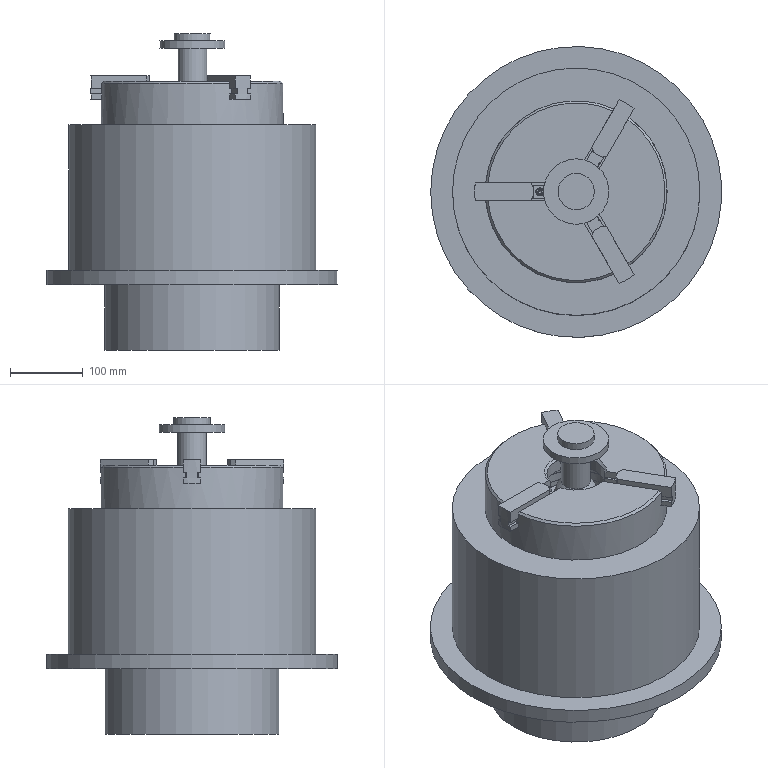Assembly | NX | mm | 45 component files | 45 solids | 1209 faces | box 400 x 400 x 435.36 mm | volume 17965879 mm3 | plane 635 | cone 295 | cylinder 211 | torus 64 | sphere 2 | spline 1 | other 1 | commonest cylinder face diameters 5 x24 6.619 x16 13 x16 6.8 x16 9 x16 15 x16 4.891 x16 10 x16
Bill of materials:
unnamed part 1 | 1 |  | Hollow cylindrical tube with a single wide, thin circular flange around it, set toward one end; the flange has a ring of evenly spaced holes.
GB-T70.1-2000,M8x20 | 8 |  | Hexagon Socket Head Cap Screw, GB-T 70.1-2000,M8x20
unnamed part 2 | 1 |  | Solid stepped round pin: a small boss on top, a thin wide flange, a short neck, a larger cylindrical body, and a smaller end step at the bottom.
unnamed part 3 | 1 |  | Flat circular plate with a large central through hole, an outer ring of 8 holes, an inner ring of 8 smaller holes, and a shallow narrower step (spigot) on one face.
unnamed part 4 | 1 |  | Flanged cup-shaped housing: a wide circular flange, a raised ring on its top face, a cylindrical body below, and a recessed pocket whose floor has a smaller central through hole and several small holes.
unnamed part 5 | 1 |  | Stepped cylinder: a large cylindrical base and a smaller top boss. The boss has a central bore and three radial slots spaced about 120 degrees apart that run from the bore out to the boss edge.
unnamed part 6 | 1 |  | Plain flat ring with a rectangular cross-section, shaped like a washer.
GB-T70.1-2000,M6x25 | 8 |  | Hexagon Socket Head Cap Screw, GB-T 70.1-2000,M6x25
GB-T70.1-2000,M6x20 | 8 |  | Hexagon Socket Head Cap Screw, GB-T 70.1-2000,M6x20
unnamed part 7 | 1 |  | Thick circular disc with a central through bore, a ring of 8 through holes, and a low raised ring around the bore on one face.
unnamed part 8 | 1 |  | Ring with a slightly stepped outer surface; its top face has narrow arc-shaped grooves that look concentric or spiral and end openly.
unnamed part 9 | 1 |  | Round part with a sphere at one end, a cylindrical shank, a thin wide flange, and a short cylindrical boss at the other end.
unnamed part 10 | 1 |  | Headed round part: a larger cylindrical head with a recess that tapers or curves down to a small central hole, on top of a narrower smooth cylindrical shank.
GB-T70.1-2000,M8x60 | 8 |  | Hexagon Socket Head Cap Screw, GB-T 70.1-2000,M8x60
unnamed part 11 | 3 |  | Long prismatic block with a grooved (I- or H-like) cross-section. One end is curved as an arc; the other end has chamfered corners.
Mates:
1. concentric | drag_plate 1 edge | chuck 1 edge
2. concentric | ball_base 1 edge | chuck 1 edge
3. concentric | force_sensor 1 edge | ball_base 1 edge
4. concentric | support_base 1 edge | force_sensor 1 edge
5. concentric | sensor_plate 1 edge | ball_base 1 edge
6. concentric | linear_bearing 1 edge | sensor_plate 1 edge
7. concentric | ball_socket 1 edge | support_base 1 edge
8. touch align | jaw 3 face | chuck 1 face
9. center | jaw 3 face | jaw 3 face | chuck 1 face | chuck 1 face
10. bond | chuck 1 component | assembly component
11. bond | jaw 3 component | assembly component
12. bond | jaw 2 component | assembly component
13. bond | jaw 1 component | assembly component
14. circular | assembly datumaxis | assembly cartesiancoordinatesystem | assembly cartesiancoordinatesystem | assembly cartesiancoordinatesystem
15. concentric | screw_plate 1 edge | chuck 1 edge
16. touch align | ball_mount 1 face | ball_socket 1 face
17. bond | ball_base 1 component | assembly component
18. bond | screw_m8x20 8 component | assembly component
19. bond | screw_m8x20 7 component | assembly component
20. bond | screw_m8x20 6 component | assembly component
21. circular | assembly datumaxis | assembly cartesiancoordinatesystem | assembly cartesiancoordinatesystem | assembly cartesiancoordinatesystem | assembly cartesiancoordinatesystem | assembly cartesiancoordinatesystem | assembly cartesiancoordinatesystem | assembly cartesiancoordinatesystem | assembly cartesiancoordinatesystem
22. bond | screw_m8x20 5 component | assembly component
23. bond | screw_m8x20 4 component | assembly component
24. bond | screw_m8x20 3 component | assembly component
25. bond | screw_m8x20 2 component | assembly component
26. bond | screw_m8x20 1 component | assembly component
27. bond | sensor_plate 1 component | assembly component
28. bond | screw_m6x20 8 component | assembly component
29. bond | screw_m6x20 7 component | assembly component
30. bond | screw_m6x20 6 component | assembly component
31. bond | screw_m6x20 5 component | assembly component
32. bond | screw_m6x20 4 component | assembly component
33. bond | screw_m6x20 3 component | assembly component
34. bond | screw_m6x20 2 component | assembly component
35. bond | screw_m6x20 1 component | assembly component
36. circular | assembly datumaxis | assembly cartesiancoordinatesystem | assembly cartesiancoordinatesystem | assembly cartesiancoordinatesystem | assembly cartesiancoordinatesystem | assembly cartesiancoordinatesystem | assembly cartesiancoordinatesystem | assembly cartesiancoordinatesystem | assembly cartesiancoordinatesystem
37. bond | linear_bearing 1 component | assembly component
38. bond | screw_m6x25 8 component | assembly component
39. bond | screw_m6x25 7 component | assembly component
40. bond | screw_m6x25 6 component | assembly component
41. bond | screw_m6x25 5 component | assembly component
42. bond | screw_m6x25 4 component | assembly component
43. bond | screw_m6x25 3 component | assembly component
44. bond | screw_m6x25 2 component | assembly component
45. bond | screw_m6x25 1 component | assembly component
46. circular | assembly datumaxis | assembly cartesiancoordinatesystem | assembly cartesiancoordinatesystem | assembly cartesiancoordinatesystem | assembly cartesiancoordinatesystem | assembly cartesiancoordinatesystem | assembly cartesiancoordinatesystem | assembly cartesiancoordinatesystem | assembly cartesiancoordinatesystem
47. bond | support_base 1 component | assembly component
48. bond | screw_m8x60 8 component | assembly component
49. bond | screw_m8x60 7 component | assembly component
50. bond | screw_m8x60 6 component | assembly component
51. bond | screw_m8x60 5 component | assembly component
52. bond | screw_m8x60 4 component | assembly component
53. bond | screw_m8x60 3 component | assembly component
54. bond | screw_m8x60 2 component | assembly component
55. bond | screw_m8x60 1 component | assembly component
56. circular | assembly datumaxis | assembly cartesiancoordinatesystem | assembly cartesiancoordinatesystem | assembly cartesiancoordinatesystem | assembly cartesiancoordinatesystem | assembly cartesiancoordinatesystem | assembly cartesiancoordinatesystem | assembly cartesiancoordinatesystem | assembly cartesiancoordinatesystem